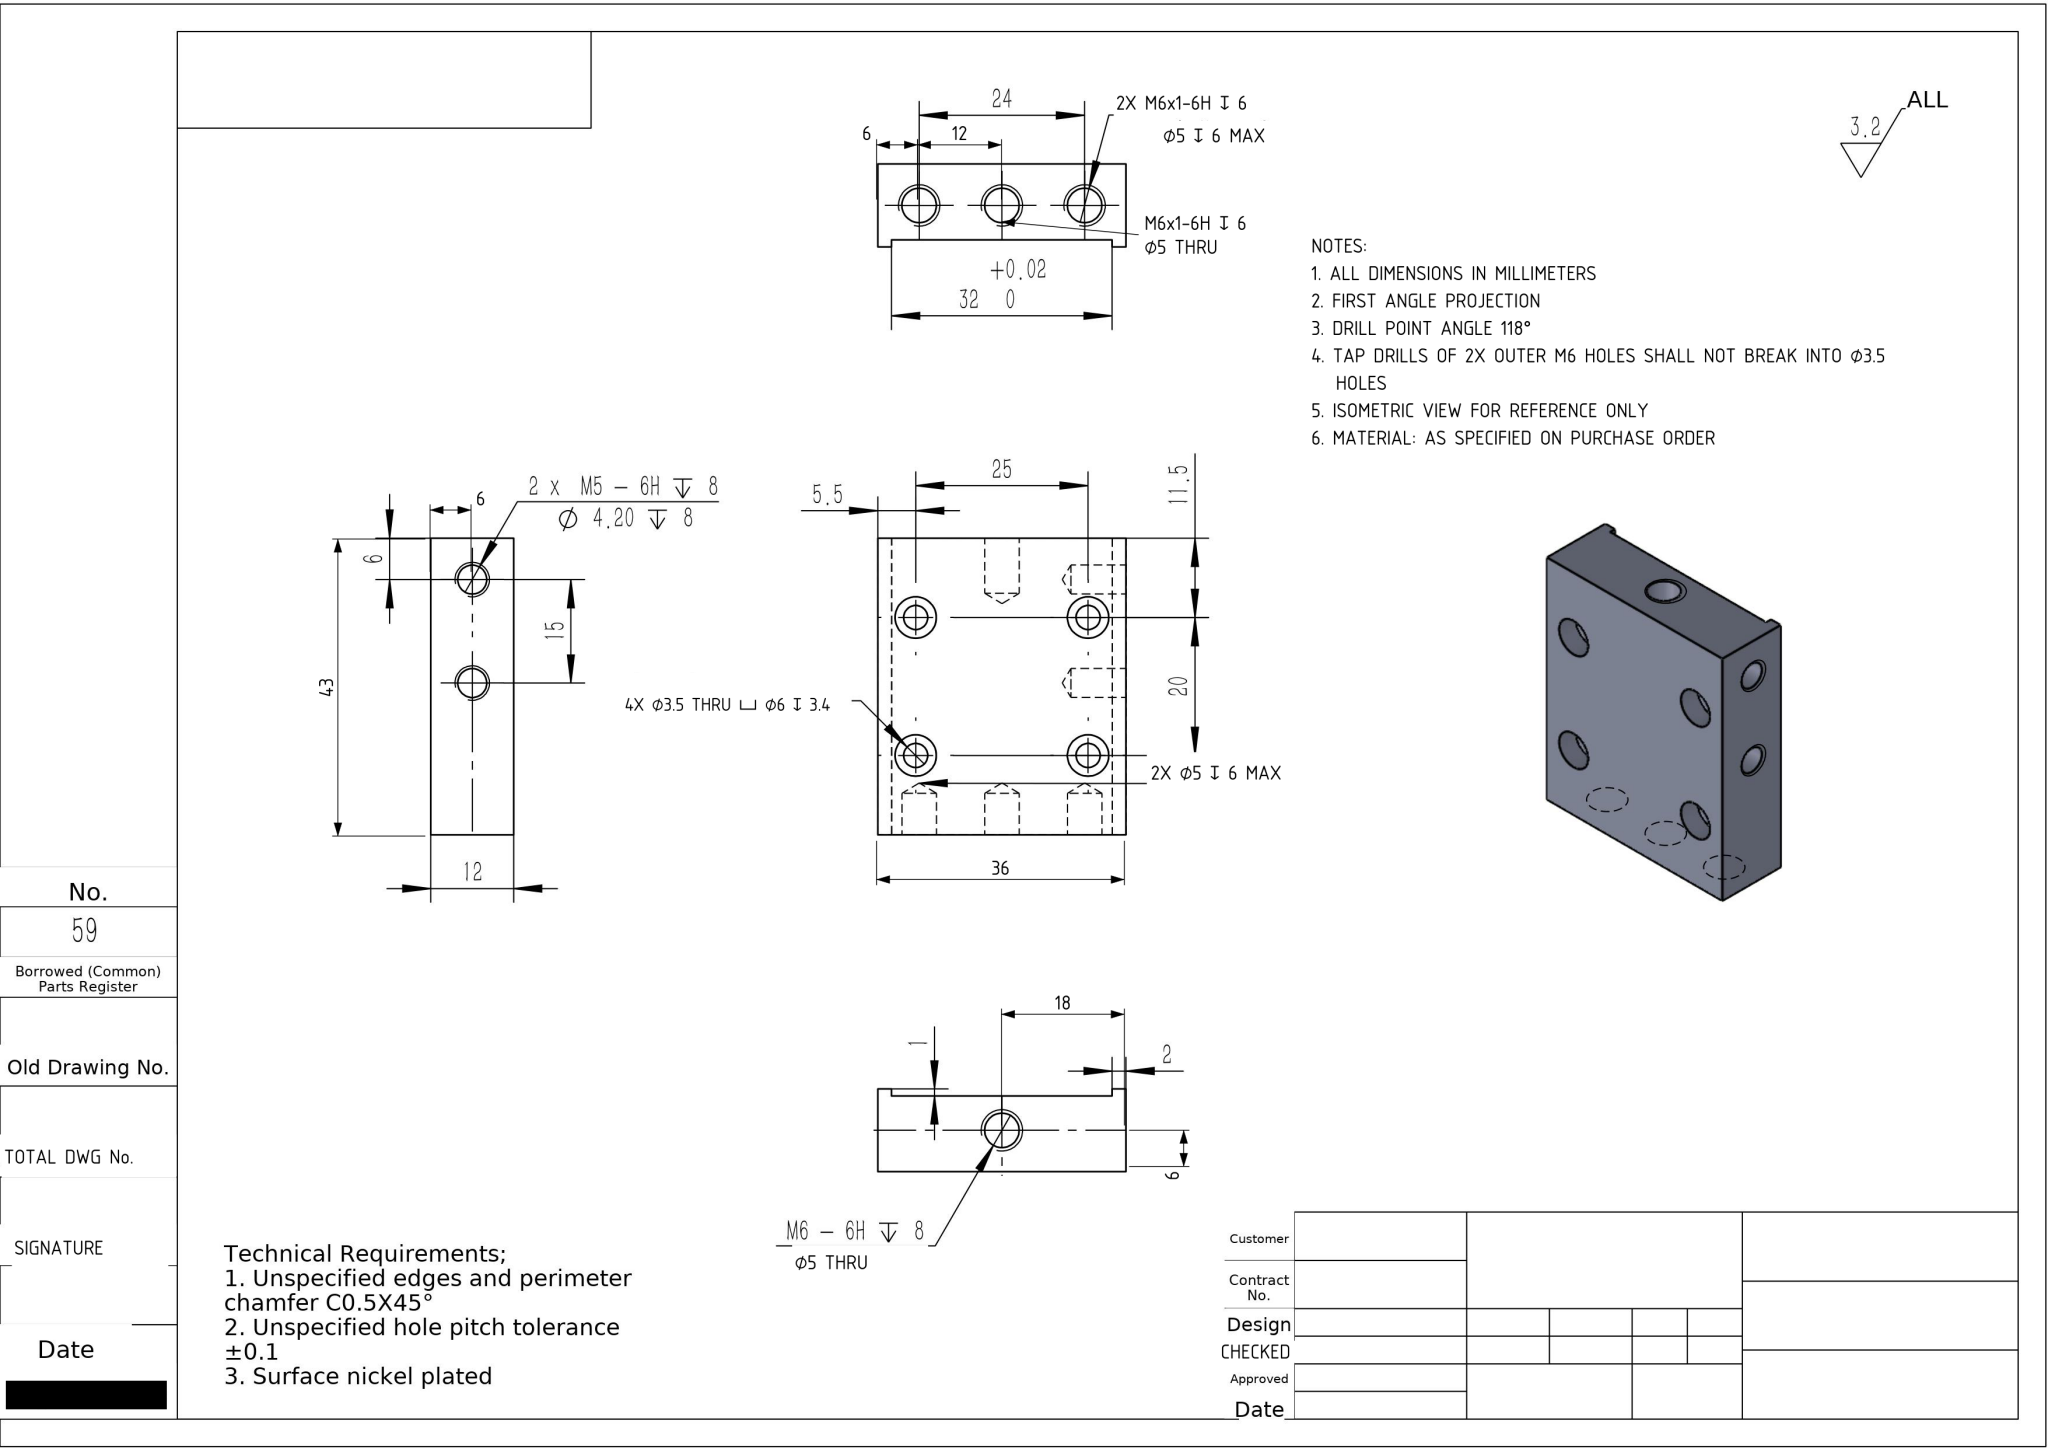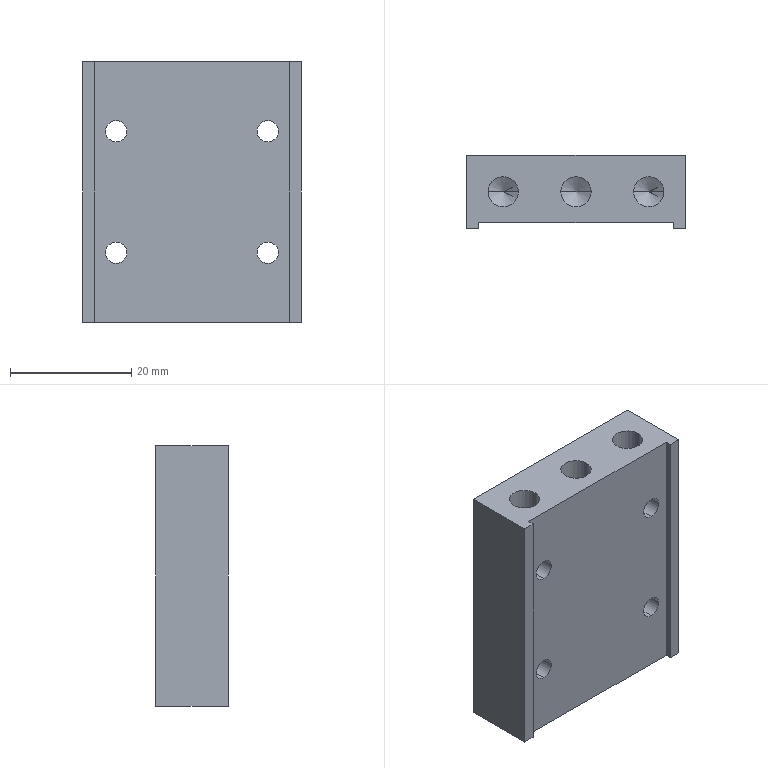Part | NX | mm | 1 solid | 54 faces | box 36 x 12 x 43 mm | volume 15740 mm3 | cylinder 28 | plane 14 | cone 12 | commonest cylinder face diameters 5 x8 6 x8 3.5 x8 4.2 x4